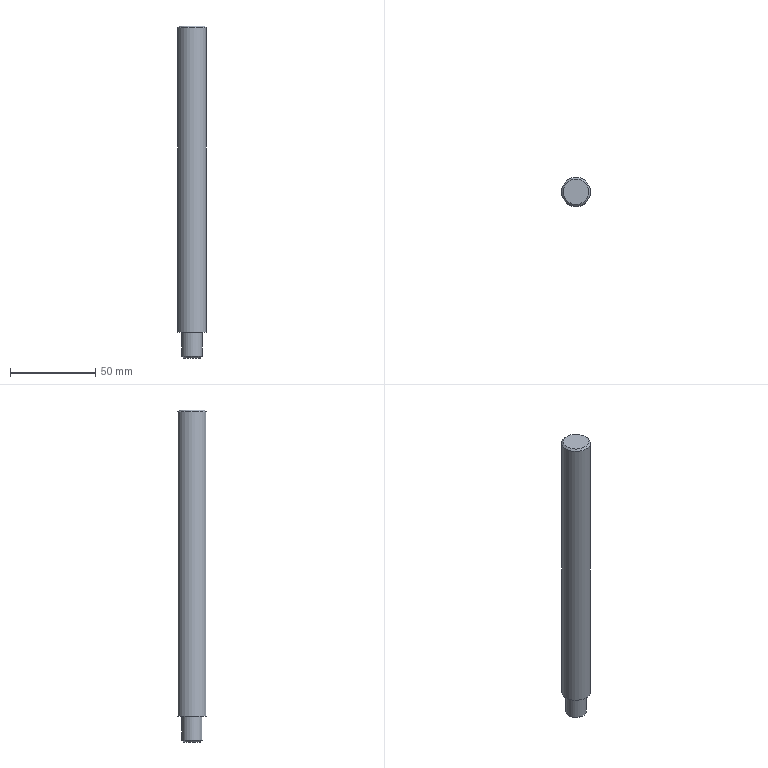Component | NX | EJECTOR_PIN | 1 solid | 7 faces | box 17 x 17 x 195 mm | volume 42509 mm3 | plane 3 | cylinder 2 | cone 2 | commonest cylinder face diameters 12 x1 17 x1
STEP:
#1=CARTESIAN_POINT('',(0.,0.,0.));
#2=DIRECTION('',(0.,0.,1.));
#3=DIRECTION('',(1.,0.,0.));
#4=AXIS2_PLACEMENT_3D('',#1,#2,#3);
#5=CARTESIAN_POINT('',(-5.,-7.5,198.));
#6=VERTEX_POINT('',#5);
#7=CARTESIAN_POINT('',(-0.,-7.5,198.));
#8=DIRECTION('',(0.,0.,-1.));
#9=DIRECTION('',(-1.,0.,0.));
#10=AXIS2_PLACEMENT_3D('',#7,#8,#9);
#11=CIRCLE('',#10,5.);
#12=CARTESIAN_POINT('',(-0.,-7.5,198.));
#13=DIRECTION('',(0.,0.,-1.));
#14=DIRECTION('',(-1.,0.,0.));
#15=AXIS2_PLACEMENT_3D('',#12,#13,#14);
#16=PLANE('',#15);
#17=CARTESIAN_POINT('',(0.,0.));
#18=DIRECTION('',(1.,0.));
#19=AXIS2_PLACEMENT_2D('',#17,#18);
#20=CIRCLE('',#19,5.);
#21=(GEOMETRIC_REPRESENTATION_CONTEXT(2)PARAMETRIC_REPRESENTATION_CONTEXT()REPRESENTATION_CONTEXT('',''));
#22=DEFINITIONAL_REPRESENTATION('',(#20),#21);
#23=PCURVE('',#16,#22);
#24=CARTESIAN_POINT('',(-0.,-7.5,199.));
#25=DIRECTION('',(0.,0.,1.));
#26=DIRECTION('',(1.,0.,0.));
#27=AXIS2_PLACEMENT_3D('',#24,#25,#26);
#28=CONICAL_SURFACE('',#27,6.,0.7854);
#29=CARTESIAN_POINT('',(9.425,-1.));
#30=DIRECTION('',(-1.,0.));
#31=VECTOR('',#30,1.);
#32=LINE('',#29,#31);
#33=(GEOMETRIC_REPRESENTATION_CONTEXT(2)PARAMETRIC_REPRESENTATION_CONTEXT()REPRESENTATION_CONTEXT('',''));
#34=DEFINITIONAL_REPRESENTATION('',(#32),#33);
#35=PCURVE('',#28,#34);
#36=SURFACE_CURVE('',#11,(#23,#35),.PCURVE_S1.);
#37=EDGE_CURVE('',#6,#6,#36,.T.);
#38=ORIENTED_EDGE('',*,*,#37,.T.);
#39=EDGE_LOOP('',(#38));
#40=FACE_BOUND('',#39,.T.);
#41=ADVANCED_FACE('',(#40),#16,.T.);
#42=CARTESIAN_POINT('',(-6.,-7.5,199.));
#43=VERTEX_POINT('',#42);
#44=CARTESIAN_POINT('',(6.,-7.5,199.));
#45=VERTEX_POINT('',#44);
#46=CARTESIAN_POINT('',(-0.,-7.5,199.));
#47=DIRECTION('',(0.,0.,1.));
#48=DIRECTION('',(-1.,0.,0.));
#49=AXIS2_PLACEMENT_3D('',#46,#47,#48);
#50=CIRCLE('',#49,6.);
#51=CARTESIAN_POINT('',(-0.,-7.5,198.));
#52=DIRECTION('',(0.,0.,1.));
#53=DIRECTION('',(1.,0.,0.));
#54=AXIS2_PLACEMENT_3D('',#51,#52,#53);
#55=CYLINDRICAL_SURFACE('',#54,6.);
#56=CARTESIAN_POINT('',(3.142,1.));
#57=DIRECTION('',(1.,0.));
#58=VECTOR('',#57,1.);
#59=LINE('',#56,#58);
#60=(GEOMETRIC_REPRESENTATION_CONTEXT(2)PARAMETRIC_REPRESENTATION_CONTEXT()REPRESENTATION_CONTEXT('',''));
#61=DEFINITIONAL_REPRESENTATION('',(#59),#60);
#62=PCURVE('',#55,#61);
#63=CARTESIAN_POINT('',(3.142,0.));
#64=DIRECTION('',(1.,0.));
#65=VECTOR('',#64,1.);
#66=LINE('',#63,#65);
#67=(GEOMETRIC_REPRESENTATION_CONTEXT(2)PARAMETRIC_REPRESENTATION_CONTEXT()REPRESENTATION_CONTEXT('',''));
#68=DEFINITIONAL_REPRESENTATION('',(#66),#67);
#69=PCURVE('',#28,#68);
#70=SURFACE_CURVE('',#50,(#62,#69),.PCURVE_S1.);
#71=EDGE_CURVE('',#43,#45,#70,.T.);
#72=ORIENTED_EDGE('',*,*,#71,.T.);
#73=CARTESIAN_POINT('',(6.,-7.5,213.));
#74=VERTEX_POINT('',#73);
#75=CARTESIAN_POINT('',(6.,-7.5,199.));
#76=CARTESIAN_POINT('',(6.,-7.5,213.));
#77=B_SPLINE_CURVE_WITH_KNOTS('',1,(#75,#76),.UNSPECIFIED.,.F.,.F.,(2,2),(1.,15.),.PIECEWISE_BEZIER_KNOTS.);
#78=CARTESIAN_POINT('',(6.283,0.));
#79=DIRECTION('',(0.,1.));
#80=VECTOR('',#79,1.);
#81=LINE('',#78,#80);
#82=(GEOMETRIC_REPRESENTATION_CONTEXT(2)PARAMETRIC_REPRESENTATION_CONTEXT()REPRESENTATION_CONTEXT('',''));
#83=DEFINITIONAL_REPRESENTATION('',(#81),#82);
#84=PCURVE('',#55,#83);
#85=CARTESIAN_POINT('',(0.,0.));
#86=DIRECTION('',(0.,1.));
#87=VECTOR('',#86,1.);
#88=LINE('',#85,#87);
#89=(GEOMETRIC_REPRESENTATION_CONTEXT(2)PARAMETRIC_REPRESENTATION_CONTEXT()REPRESENTATION_CONTEXT('',''));
#90=DEFINITIONAL_REPRESENTATION('',(#88),#89);
#91=PCURVE('',#55,#90);
#92=SEAM_CURVE('',#77,(#84,#91),.PCURVE_S1.);
#93=EDGE_CURVE('',#45,#74,#92,.T.);
#94=ORIENTED_EDGE('',*,*,#93,.T.);
#95=CARTESIAN_POINT('',(-0.,-7.5,213.));
#96=DIRECTION('',(0.,0.,-1.));
#97=DIRECTION('',(1.,0.,0.));
#98=AXIS2_PLACEMENT_3D('',#95,#96,#97);
#99=CIRCLE('',#98,6.);
#100=CARTESIAN_POINT('',(6.283,15.));
#101=DIRECTION('',(-1.,0.));
#102=VECTOR('',#101,1.);
#103=LINE('',#100,#102);
#104=(GEOMETRIC_REPRESENTATION_CONTEXT(2)PARAMETRIC_REPRESENTATION_CONTEXT()REPRESENTATION_CONTEXT('',''));
#105=DEFINITIONAL_REPRESENTATION('',(#103),#104);
#106=PCURVE('',#55,#105);
#107=CARTESIAN_POINT('',(-0.,-7.5,213.));
#108=DIRECTION('',(0.,0.,-1.));
#109=DIRECTION('',(-1.,0.,0.));
#110=AXIS2_PLACEMENT_3D('',#107,#108,#109);
#111=PLANE('',#110);
#112=CARTESIAN_POINT('',(0.,0.));
#113=DIRECTION('',(-1.,0.));
#114=AXIS2_PLACEMENT_2D('',#112,#113);
#115=CIRCLE('',#114,6.);
#116=(GEOMETRIC_REPRESENTATION_CONTEXT(2)PARAMETRIC_REPRESENTATION_CONTEXT()REPRESENTATION_CONTEXT('',''));
#117=DEFINITIONAL_REPRESENTATION('',(#115),#116);
#118=PCURVE('',#111,#117);
#119=SURFACE_CURVE('',#99,(#106,#118),.PCURVE_S1.);
#120=EDGE_CURVE('',#74,#74,#119,.T.);
#121=ORIENTED_EDGE('',*,*,#120,.T.);
#122=ORIENTED_EDGE('',*,*,#93,.F.);
#123=CARTESIAN_POINT('',(-0.,-7.5,199.));
#124=DIRECTION('',(0.,0.,1.));
#125=DIRECTION('',(-1.,0.,0.));
#126=AXIS2_PLACEMENT_3D('',#123,#124,#125);
#127=CIRCLE('',#126,6.);
#128=CARTESIAN_POINT('',(-3.142,1.));
#129=DIRECTION('',(1.,0.));
#130=VECTOR('',#129,1.);
#131=LINE('',#128,#130);
#132=(GEOMETRIC_REPRESENTATION_CONTEXT(2)PARAMETRIC_REPRESENTATION_CONTEXT()REPRESENTATION_CONTEXT('',''));
#133=DEFINITIONAL_REPRESENTATION('',(#131),#132);
#134=PCURVE('',#55,#133);
#135=CARTESIAN_POINT('',(3.142,0.));
#136=DIRECTION('',(1.,0.));
#137=VECTOR('',#136,1.);
#138=LINE('',#135,#137);
#139=(GEOMETRIC_REPRESENTATION_CONTEXT(2)PARAMETRIC_REPRESENTATION_CONTEXT()REPRESENTATION_CONTEXT('',''));
#140=DEFINITIONAL_REPRESENTATION('',(#138),#139);
#141=PCURVE('',#28,#140);
#142=SURFACE_CURVE('',#127,(#134,#141),.PCURVE_S1.);
#143=EDGE_CURVE('',#45,#43,#142,.T.);
#144=ORIENTED_EDGE('',*,*,#143,.T.);
#145=EDGE_LOOP('',(#72,#94,#121,#122,#144));
#146=FACE_BOUND('',#145,.T.);
#147=ADVANCED_FACE('',(#146),#55,.T.);
#148=CARTESIAN_POINT('',(7.5,-7.5,393.));
#149=VERTEX_POINT('',#148);
#150=CARTESIAN_POINT('',(-0.,-7.5,393.));
#151=DIRECTION('',(0.,0.,1.));
#152=DIRECTION('',(1.,0.,0.));
#153=AXIS2_PLACEMENT_3D('',#150,#151,#152);
#154=CIRCLE('',#153,7.5);
#155=CARTESIAN_POINT('',(-0.,-7.5,393.));
#156=DIRECTION('',(0.,0.,1.));
#157=DIRECTION('',(1.,0.,0.));
#158=AXIS2_PLACEMENT_3D('',#155,#156,#157);
#159=PLANE('',#158);
#160=CARTESIAN_POINT('',(0.,0.));
#161=DIRECTION('',(1.,0.));
#162=AXIS2_PLACEMENT_2D('',#160,#161);
#163=CIRCLE('',#162,7.5);
#164=(GEOMETRIC_REPRESENTATION_CONTEXT(2)PARAMETRIC_REPRESENTATION_CONTEXT()REPRESENTATION_CONTEXT('',''));
#165=DEFINITIONAL_REPRESENTATION('',(#163),#164);
#166=PCURVE('',#159,#165);
#167=CARTESIAN_POINT('',(-0.,-7.5,392.));
#168=DIRECTION('',(0.,0.,-1.));
#169=DIRECTION('',(-1.,0.,0.));
#170=AXIS2_PLACEMENT_3D('',#167,#168,#169);
#171=CONICAL_SURFACE('',#170,8.5,0.7854);
#172=CARTESIAN_POINT('',(9.425,-1.));
#173=DIRECTION('',(-1.,0.));
#174=VECTOR('',#173,1.);
#175=LINE('',#172,#174);
#176=(GEOMETRIC_REPRESENTATION_CONTEXT(2)PARAMETRIC_REPRESENTATION_CONTEXT()REPRESENTATION_CONTEXT('',''));
#177=DEFINITIONAL_REPRESENTATION('',(#175),#176);
#178=PCURVE('',#171,#177);
#179=SURFACE_CURVE('',#154,(#166,#178),.PCURVE_S1.);
#180=EDGE_CURVE('',#149,#149,#179,.T.);
#181=ORIENTED_EDGE('',*,*,#180,.T.);
#182=EDGE_LOOP('',(#181));
#183=FACE_BOUND('',#182,.T.);
#184=ADVANCED_FACE('',(#183),#159,.T.);
#185=ORIENTED_EDGE('',*,*,#120,.F.);
#186=EDGE_LOOP('',(#185));
#187=FACE_BOUND('',#186,.T.);
#188=CARTESIAN_POINT('',(8.5,-7.5,213.));
#189=VERTEX_POINT('',#188);
#190=CARTESIAN_POINT('',(-0.,-7.5,213.));
#191=DIRECTION('',(0.,0.,1.));
#192=DIRECTION('',(1.,0.,0.));
#193=AXIS2_PLACEMENT_3D('',#190,#191,#192);
#194=CIRCLE('',#193,8.5);
#195=CARTESIAN_POINT('',(-8.5,0.));
#196=CARTESIAN_POINT('',(-8.5,14.722));
#197=CARTESIAN_POINT('',(4.25,7.361));
#198=CARTESIAN_POINT('',(17.,0.));
#199=CARTESIAN_POINT('',(4.25,-7.361));
#200=CARTESIAN_POINT('',(-8.5,-14.722));
#201=CARTESIAN_POINT('',(-8.5,0.));
#202=(BOUNDED_CURVE()B_SPLINE_CURVE(2,(#195,#196,#197,#198,#199,#200,#201),.UNSPECIFIED.,.T.,.F.)B_SPLINE_CURVE_WITH_KNOTS((1,2,2,2,2,1),(-2.094,0.,2.094,4.189,6.283,8.378),.UNSPECIFIED.)CURVE()GEOMETRIC_REPRESENTATION_ITEM()RATIONAL_B_SPLINE_CURVE((1.,0.5,1.,0.5,1.,0.5,1.))REPRESENTATION_ITEM(''));
#203=(GEOMETRIC_REPRESENTATION_CONTEXT(2)PARAMETRIC_REPRESENTATION_CONTEXT()REPRESENTATION_CONTEXT('',''));
#204=DEFINITIONAL_REPRESENTATION('',(#202),#203);
#205=PCURVE('',#111,#204);
#206=CARTESIAN_POINT('',(-0.,-7.5,213.));
#207=DIRECTION('',(0.,0.,1.));
#208=DIRECTION('',(1.,0.,0.));
#209=AXIS2_PLACEMENT_3D('',#206,#207,#208);
#210=CYLINDRICAL_SURFACE('',#209,8.5);
#211=CARTESIAN_POINT('',(0.,0.));
#212=DIRECTION('',(1.,0.));
#213=VECTOR('',#212,1.);
#214=LINE('',#211,#213);
#215=(GEOMETRIC_REPRESENTATION_CONTEXT(2)PARAMETRIC_REPRESENTATION_CONTEXT()REPRESENTATION_CONTEXT('',''));
#216=DEFINITIONAL_REPRESENTATION('',(#214),#215);
#217=PCURVE('',#210,#216);
#218=SURFACE_CURVE('',#194,(#205,#217),.PCURVE_S1.);
#219=EDGE_CURVE('',#189,#189,#218,.T.);
#220=ORIENTED_EDGE('',*,*,#219,.F.);
#221=EDGE_LOOP('',(#220));
#222=FACE_BOUND('',#221,.T.);
#223=ADVANCED_FACE('',(#187,#222),#111,.T.);
#224=CARTESIAN_POINT('',(8.5,-7.5,392.));
#225=VERTEX_POINT('',#224);
#226=CARTESIAN_POINT('',(-0.,-7.5,392.));
#227=DIRECTION('',(0.,0.,-1.));
#228=DIRECTION('',(1.,0.,0.));
#229=AXIS2_PLACEMENT_3D('',#226,#227,#228);
#230=CIRCLE('',#229,8.5);
#231=CARTESIAN_POINT('',(6.283,179.));
#232=DIRECTION('',(-1.,0.));
#233=VECTOR('',#232,1.);
#234=LINE('',#231,#233);
#235=(GEOMETRIC_REPRESENTATION_CONTEXT(2)PARAMETRIC_REPRESENTATION_CONTEXT()REPRESENTATION_CONTEXT('',''));
#236=DEFINITIONAL_REPRESENTATION('',(#234),#235);
#237=PCURVE('',#210,#236);
#238=CARTESIAN_POINT('',(3.142,0.));
#239=DIRECTION('',(1.,0.));
#240=VECTOR('',#239,1.);
#241=LINE('',#238,#240);
#242=(GEOMETRIC_REPRESENTATION_CONTEXT(2)PARAMETRIC_REPRESENTATION_CONTEXT()REPRESENTATION_CONTEXT('',''));
#243=DEFINITIONAL_REPRESENTATION('',(#241),#242);
#244=PCURVE('',#171,#243);
#245=SURFACE_CURVE('',#230,(#237,#244),.PCURVE_S1.);
#246=EDGE_CURVE('',#225,#225,#245,.T.);
#247=ORIENTED_EDGE('',*,*,#246,.T.);
#248=CARTESIAN_POINT('',(8.5,-7.5,213.));
#249=CARTESIAN_POINT('',(8.5,-7.5,392.));
#250=B_SPLINE_CURVE_WITH_KNOTS('',1,(#248,#249),.UNSPECIFIED.,.F.,.F.,(2,2),(0.,179.),.PIECEWISE_BEZIER_KNOTS.);
#251=CARTESIAN_POINT('',(0.,0.));
#252=DIRECTION('',(0.,1.));
#253=VECTOR('',#252,1.);
#254=LINE('',#251,#253);
#255=(GEOMETRIC_REPRESENTATION_CONTEXT(2)PARAMETRIC_REPRESENTATION_CONTEXT()REPRESENTATION_CONTEXT('',''));
#256=DEFINITIONAL_REPRESENTATION('',(#254),#255);
#257=PCURVE('',#210,#256);
#258=CARTESIAN_POINT('',(6.283,0.));
#259=DIRECTION('',(0.,1.));
#260=VECTOR('',#259,1.);
#261=LINE('',#258,#260);
#262=(GEOMETRIC_REPRESENTATION_CONTEXT(2)PARAMETRIC_REPRESENTATION_CONTEXT()REPRESENTATION_CONTEXT('',''));
#263=DEFINITIONAL_REPRESENTATION('',(#261),#262);
#264=PCURVE('',#210,#263);
#265=SEAM_CURVE('',#250,(#257,#264),.PCURVE_S1.);
#266=EDGE_CURVE('',#189,#225,#265,.T.);
#267=ORIENTED_EDGE('',*,*,#266,.F.);
#268=ORIENTED_EDGE('',*,*,#219,.T.);
#269=ORIENTED_EDGE('',*,*,#266,.T.);
#270=EDGE_LOOP('',(#247,#267,#268,#269));
#271=FACE_BOUND('',#270,.T.);
#272=ADVANCED_FACE('',(#271),#210,.T.);
#273=ORIENTED_EDGE('',*,*,#180,.F.);
#274=CARTESIAN_POINT('',(7.5,-7.5,393.));
#275=CARTESIAN_POINT('',(8.5,-7.5,392.));
#276=B_SPLINE_CURVE_WITH_KNOTS('',1,(#274,#275),.UNSPECIFIED.,.F.,.F.,(2,2),(-1.414,0.),.PIECEWISE_BEZIER_KNOTS.);
#277=CARTESIAN_POINT('',(9.425,0.));
#278=DIRECTION('',(0.,1.));
#279=VECTOR('',#278,1.);
#280=LINE('',#277,#279);
#281=(GEOMETRIC_REPRESENTATION_CONTEXT(2)PARAMETRIC_REPRESENTATION_CONTEXT()REPRESENTATION_CONTEXT('',''));
#282=DEFINITIONAL_REPRESENTATION('',(#280),#281);
#283=PCURVE('',#171,#282);
#284=CARTESIAN_POINT('',(3.142,0.));
#285=DIRECTION('',(0.,1.));
#286=VECTOR('',#285,1.);
#287=LINE('',#284,#286);
#288=(GEOMETRIC_REPRESENTATION_CONTEXT(2)PARAMETRIC_REPRESENTATION_CONTEXT()REPRESENTATION_CONTEXT('',''));
#289=DEFINITIONAL_REPRESENTATION('',(#287),#288);
#290=PCURVE('',#171,#289);
#291=SEAM_CURVE('',#276,(#283,#290),.PCURVE_S1.);
#292=EDGE_CURVE('',#149,#225,#291,.T.);
#293=ORIENTED_EDGE('',*,*,#292,.T.);
#294=ORIENTED_EDGE('',*,*,#246,.F.);
#295=ORIENTED_EDGE('',*,*,#292,.F.);
#296=EDGE_LOOP('',(#273,#293,#294,#295));
#297=FACE_BOUND('',#296,.T.);
#298=ADVANCED_FACE('',(#297),#171,.T.);
#299=ORIENTED_EDGE('',*,*,#37,.F.);
#300=CARTESIAN_POINT('',(-5.,-7.5,198.));
#301=CARTESIAN_POINT('',(-6.,-7.5,199.));
#302=B_SPLINE_CURVE_WITH_KNOTS('',1,(#300,#301),.UNSPECIFIED.,.F.,.F.,(2,2),(-1.414,0.),.PIECEWISE_BEZIER_KNOTS.);
#303=CARTESIAN_POINT('',(9.425,0.));
#304=DIRECTION('',(0.,1.));
#305=VECTOR('',#304,1.);
#306=LINE('',#303,#305);
#307=(GEOMETRIC_REPRESENTATION_CONTEXT(2)PARAMETRIC_REPRESENTATION_CONTEXT()REPRESENTATION_CONTEXT('',''));
#308=DEFINITIONAL_REPRESENTATION('',(#306),#307);
#309=PCURVE('',#28,#308);
#310=CARTESIAN_POINT('',(3.142,0.));
#311=DIRECTION('',(0.,1.));
#312=VECTOR('',#311,1.);
#313=LINE('',#310,#312);
#314=(GEOMETRIC_REPRESENTATION_CONTEXT(2)PARAMETRIC_REPRESENTATION_CONTEXT()REPRESENTATION_CONTEXT('',''));
#315=DEFINITIONAL_REPRESENTATION('',(#313),#314);
#316=PCURVE('',#28,#315);
#317=SEAM_CURVE('',#302,(#309,#316),.PCURVE_S1.);
#318=EDGE_CURVE('',#6,#43,#317,.T.);
#319=ORIENTED_EDGE('',*,*,#318,.T.);
#320=ORIENTED_EDGE('',*,*,#143,.F.);
#321=ORIENTED_EDGE('',*,*,#71,.F.);
#322=ORIENTED_EDGE('',*,*,#318,.F.);
#323=EDGE_LOOP('',(#299,#319,#320,#321,#322));
#324=FACE_BOUND('',#323,.T.);
#325=ADVANCED_FACE('',(#324),#28,.T.);
#326=CLOSED_SHELL('',(#41,#147,#184,#223,#272,#298,#325));
#327=MANIFOLD_SOLID_BREP('',#326);
#328=(LENGTH_UNIT()NAMED_UNIT(*)SI_UNIT(.MILLI.,.METRE.));
#329=UNCERTAINTY_MEASURE_WITH_UNIT(LENGTH_MEASURE(0.00001),#328,'','');
#330=(NAMED_UNIT(*)PLANE_ANGLE_UNIT()SI_UNIT($,.RADIAN.));
#331=(NAMED_UNIT(*)SI_UNIT($,.STERADIAN.)SOLID_ANGLE_UNIT());
#332=(GEOMETRIC_REPRESENTATION_CONTEXT(3)GLOBAL_UNCERTAINTY_ASSIGNED_CONTEXT((#329))GLOBAL_UNIT_ASSIGNED_CONTEXT((#328,#330,#331))REPRESENTATION_CONTEXT('',''));
#333=ADVANCED_BREP_SHAPE_REPRESENTATION('',(#4,#327),#332);